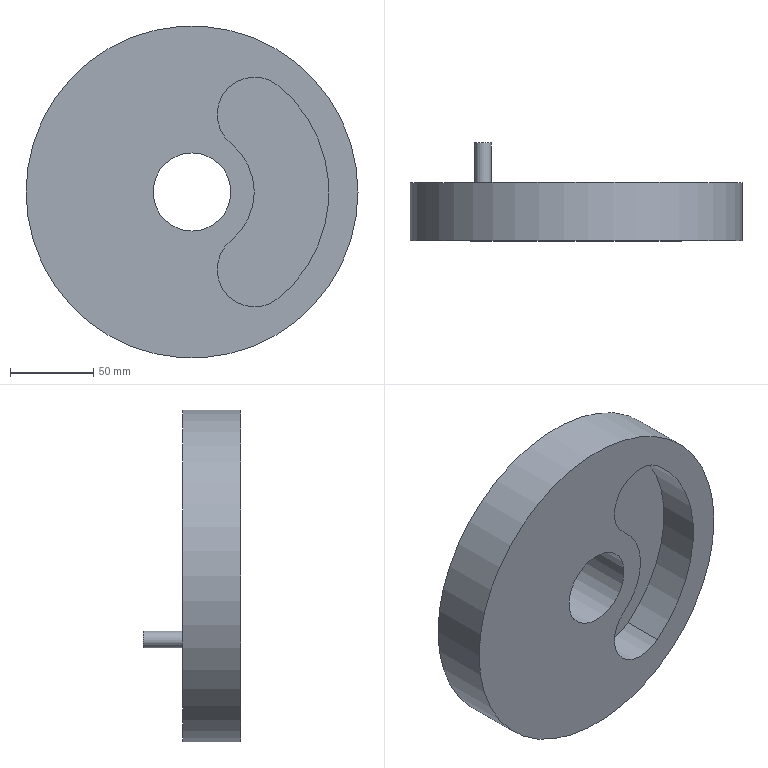Component | NX | TURNTABLE | 1 solid | 11 faces | box 200 x 59 x 200 mm | volume 880594 mm3 | cylinder 7 | plane 4 | commonest cylinder face diameters 45 x2 165 x1 47 x1 200 x1 75 x1 10 x1
STEP:
#1=CARTESIAN_POINT('',(0.,0.,0.));
#2=DIRECTION('',(0.,0.,1.));
#3=DIRECTION('',(1.,0.,0.));
#4=AXIS2_PLACEMENT_3D('',#1,#2,#3);
#5=CARTESIAN_POINT('',(23.557,-35.,29.178));
#6=VERTEX_POINT('',#5);
#7=CARTESIAN_POINT('',(23.557,-10.,29.178));
#8=VERTEX_POINT('',#7);
#9=CARTESIAN_POINT('',(23.557,-35.,29.178));
#10=DIRECTION('',(0.,1.,0.));
#11=VECTOR('',#10,1.);
#12=LINE('',#9,#11);
#13=CARTESIAN_POINT('',(37.691,-35.,46.684));
#14=DIRECTION('',(0.,1.,0.));
#15=DIRECTION('',(0.,0.,1.));
#16=AXIS2_PLACEMENT_3D('',#13,#14,#15);
#17=CYLINDRICAL_SURFACE('',#16,22.5);
#18=CARTESIAN_POINT('',(3.821,0.));
#19=DIRECTION('',(0.,1.));
#20=VECTOR('',#19,1.);
#21=LINE('',#18,#20);
#22=(GEOMETRIC_REPRESENTATION_CONTEXT(2)PARAMETRIC_REPRESENTATION_CONTEXT()REPRESENTATION_CONTEXT('',''));
#23=DEFINITIONAL_REPRESENTATION('',(#21),#22);
#24=PCURVE('',#17,#23);
#25=CARTESIAN_POINT('',(0.,-35.,0.));
#26=DIRECTION('',(0.,1.,0.));
#27=DIRECTION('',(0.,0.,1.));
#28=AXIS2_PLACEMENT_3D('',#25,#26,#27);
#29=CYLINDRICAL_SURFACE('',#28,37.5);
#30=CARTESIAN_POINT('',(0.6792,0.));
#31=DIRECTION('',(0.,1.));
#32=VECTOR('',#31,1.);
#33=LINE('',#30,#32);
#34=(GEOMETRIC_REPRESENTATION_CONTEXT(2)PARAMETRIC_REPRESENTATION_CONTEXT()REPRESENTATION_CONTEXT('',''));
#35=DEFINITIONAL_REPRESENTATION('',(#33),#34);
#36=PCURVE('',#29,#35);
#37=SURFACE_CURVE('',#12,(#24,#36),.PCURVE_S1.);
#38=EDGE_CURVE('',#6,#8,#37,.T.);
#39=ORIENTED_EDGE('',*,*,#38,.F.);
#40=CARTESIAN_POINT('',(51.825,-35.,64.191));
#41=VERTEX_POINT('',#40);
#42=CARTESIAN_POINT('',(37.691,-35.,46.684));
#43=DIRECTION('',(0.,-1.,0.));
#44=DIRECTION('',(0.7193,0.,-0.6947));
#45=AXIS2_PLACEMENT_3D('',#42,#43,#44);
#46=CIRCLE('',#45,22.5);
#47=CARTESIAN_POINT('',(8.622,0.));
#48=DIRECTION('',(-1.,0.));
#49=VECTOR('',#48,1.);
#50=LINE('',#47,#49);
#51=(GEOMETRIC_REPRESENTATION_CONTEXT(2)PARAMETRIC_REPRESENTATION_CONTEXT()REPRESENTATION_CONTEXT('',''));
#52=DEFINITIONAL_REPRESENTATION('',(#50),#51);
#53=PCURVE('',#17,#52);
#54=CARTESIAN_POINT('',(12.564,-35.,15.561));
#55=DIRECTION('',(0.,-1.,0.));
#56=DIRECTION('',(0.,0.,-1.));
#57=AXIS2_PLACEMENT_3D('',#54,#55,#56);
#58=PLANE('',#57);
#59=CARTESIAN_POINT('',(-31.123,25.127));
#60=DIRECTION('',(0.6947,0.7193));
#61=AXIS2_PLACEMENT_2D('',#59,#60);
#62=CIRCLE('',#61,22.5);
#63=(GEOMETRIC_REPRESENTATION_CONTEXT(2)PARAMETRIC_REPRESENTATION_CONTEXT()REPRESENTATION_CONTEXT('',''));
#64=DEFINITIONAL_REPRESENTATION('',(#62),#63);
#65=PCURVE('',#58,#64);
#66=SURFACE_CURVE('',#46,(#53,#65),.PCURVE_S1.);
#67=EDGE_CURVE('',#41,#6,#66,.T.);
#68=ORIENTED_EDGE('',*,*,#67,.F.);
#69=CARTESIAN_POINT('',(51.825,-10.,64.191));
#70=VERTEX_POINT('',#69);
#71=CARTESIAN_POINT('',(51.825,-35.,64.191));
#72=DIRECTION('',(0.,1.,0.));
#73=VECTOR('',#72,1.);
#74=LINE('',#71,#73);
#75=CARTESIAN_POINT('',(6.962,0.));
#76=DIRECTION('',(0.,1.));
#77=VECTOR('',#76,1.);
#78=LINE('',#75,#77);
#79=(GEOMETRIC_REPRESENTATION_CONTEXT(2)PARAMETRIC_REPRESENTATION_CONTEXT()REPRESENTATION_CONTEXT('',''));
#80=DEFINITIONAL_REPRESENTATION('',(#78),#79);
#81=PCURVE('',#17,#80);
#82=CARTESIAN_POINT('',(0.,-35.,0.));
#83=DIRECTION('',(0.,1.,0.));
#84=DIRECTION('',(0.,0.,1.));
#85=AXIS2_PLACEMENT_3D('',#82,#83,#84);
#86=CYLINDRICAL_SURFACE('',#85,82.5);
#87=CARTESIAN_POINT('',(0.6792,0.));
#88=DIRECTION('',(0.,1.));
#89=VECTOR('',#88,1.);
#90=LINE('',#87,#89);
#91=(GEOMETRIC_REPRESENTATION_CONTEXT(2)PARAMETRIC_REPRESENTATION_CONTEXT()REPRESENTATION_CONTEXT('',''));
#92=DEFINITIONAL_REPRESENTATION('',(#90),#91);
#93=PCURVE('',#86,#92);
#94=SURFACE_CURVE('',#74,(#81,#93),.PCURVE_S1.);
#95=EDGE_CURVE('',#41,#70,#94,.T.);
#96=ORIENTED_EDGE('',*,*,#95,.T.);
#97=CARTESIAN_POINT('',(37.691,-10.,46.684));
#98=DIRECTION('',(0.,-1.,0.));
#99=DIRECTION('',(0.7193,0.,-0.6947));
#100=AXIS2_PLACEMENT_3D('',#97,#98,#99);
#101=CIRCLE('',#100,22.5);
#102=CARTESIAN_POINT('',(8.622,25.));
#103=DIRECTION('',(-1.,0.));
#104=VECTOR('',#103,1.);
#105=LINE('',#102,#104);
#106=(GEOMETRIC_REPRESENTATION_CONTEXT(2)PARAMETRIC_REPRESENTATION_CONTEXT()REPRESENTATION_CONTEXT('',''));
#107=DEFINITIONAL_REPRESENTATION('',(#105),#106);
#108=PCURVE('',#17,#107);
#109=CARTESIAN_POINT('',(18.845,-10.,23.342));
#110=DIRECTION('',(0.,-1.,0.));
#111=DIRECTION('',(0.,0.,-1.));
#112=AXIS2_PLACEMENT_3D('',#109,#110,#111);
#113=PLANE('',#112);
#114=CARTESIAN_POINT('',(-23.342,18.845));
#115=DIRECTION('',(0.6947,0.7193));
#116=AXIS2_PLACEMENT_2D('',#114,#115);
#117=CIRCLE('',#116,22.5);
#118=(GEOMETRIC_REPRESENTATION_CONTEXT(2)PARAMETRIC_REPRESENTATION_CONTEXT()REPRESENTATION_CONTEXT('',''));
#119=DEFINITIONAL_REPRESENTATION('',(#117),#118);
#120=PCURVE('',#113,#119);
#121=SURFACE_CURVE('',#101,(#108,#120),.PCURVE_S1.);
#122=EDGE_CURVE('',#70,#8,#121,.T.);
#123=ORIENTED_EDGE('',*,*,#122,.T.);
#124=EDGE_LOOP('',(#39,#68,#96,#123));
#125=FACE_BOUND('',#124,.F.);
#126=ADVANCED_FACE('',(#125),#17,.F.);
#127=ORIENTED_EDGE('',*,*,#95,.F.);
#128=CARTESIAN_POINT('',(51.825,-35.,-64.191));
#129=VERTEX_POINT('',#128);
#130=CARTESIAN_POINT('',(0.,-35.,0.));
#131=DIRECTION('',(0.,-1.,0.));
#132=DIRECTION('',(1.,0.,-0.));
#133=AXIS2_PLACEMENT_3D('',#130,#131,#132);
#134=CIRCLE('',#133,82.5);
#135=CARTESIAN_POINT('',(7.854,0.));
#136=DIRECTION('',(-1.,0.));
#137=VECTOR('',#136,1.);
#138=LINE('',#135,#137);
#139=(GEOMETRIC_REPRESENTATION_CONTEXT(2)PARAMETRIC_REPRESENTATION_CONTEXT()REPRESENTATION_CONTEXT('',''));
#140=DEFINITIONAL_REPRESENTATION('',(#138),#139);
#141=PCURVE('',#86,#140);
#142=CARTESIAN_POINT('',(15.561,-12.564));
#143=DIRECTION('',(0.,1.));
#144=AXIS2_PLACEMENT_2D('',#142,#143);
#145=CIRCLE('',#144,82.5);
#146=(GEOMETRIC_REPRESENTATION_CONTEXT(2)PARAMETRIC_REPRESENTATION_CONTEXT()REPRESENTATION_CONTEXT('',''));
#147=DEFINITIONAL_REPRESENTATION('',(#145),#146);
#148=PCURVE('',#58,#147);
#149=SURFACE_CURVE('',#134,(#141,#148),.PCURVE_S1.);
#150=EDGE_CURVE('',#129,#41,#149,.T.);
#151=ORIENTED_EDGE('',*,*,#150,.F.);
#152=CARTESIAN_POINT('',(51.825,-10.,-64.191));
#153=VERTEX_POINT('',#152);
#154=CARTESIAN_POINT('',(51.825,-35.,-64.191));
#155=DIRECTION('',(0.,1.,0.));
#156=VECTOR('',#155,1.);
#157=LINE('',#154,#156);
#158=CARTESIAN_POINT('',(2.462,0.));
#159=DIRECTION('',(0.,1.));
#160=VECTOR('',#159,1.);
#161=LINE('',#158,#160);
#162=(GEOMETRIC_REPRESENTATION_CONTEXT(2)PARAMETRIC_REPRESENTATION_CONTEXT()REPRESENTATION_CONTEXT('',''));
#163=DEFINITIONAL_REPRESENTATION('',(#161),#162);
#164=PCURVE('',#86,#163);
#165=CARTESIAN_POINT('',(37.691,-35.,-46.684));
#166=DIRECTION('',(0.,1.,0.));
#167=DIRECTION('',(0.,0.,1.));
#168=AXIS2_PLACEMENT_3D('',#165,#166,#167);
#169=CYLINDRICAL_SURFACE('',#168,22.5);
#170=CARTESIAN_POINT('',(2.462,0.));
#171=DIRECTION('',(0.,1.));
#172=VECTOR('',#171,1.);
#173=LINE('',#170,#172);
#174=(GEOMETRIC_REPRESENTATION_CONTEXT(2)PARAMETRIC_REPRESENTATION_CONTEXT()REPRESENTATION_CONTEXT('',''));
#175=DEFINITIONAL_REPRESENTATION('',(#173),#174);
#176=PCURVE('',#169,#175);
#177=SURFACE_CURVE('',#157,(#164,#176),.PCURVE_S1.);
#178=EDGE_CURVE('',#129,#153,#177,.T.);
#179=ORIENTED_EDGE('',*,*,#178,.T.);
#180=CARTESIAN_POINT('',(0.,-10.,0.));
#181=DIRECTION('',(0.,-1.,0.));
#182=DIRECTION('',(1.,0.,-0.));
#183=AXIS2_PLACEMENT_3D('',#180,#181,#182);
#184=CIRCLE('',#183,82.5);
#185=CARTESIAN_POINT('',(7.854,25.));
#186=DIRECTION('',(-1.,0.));
#187=VECTOR('',#186,1.);
#188=LINE('',#185,#187);
#189=(GEOMETRIC_REPRESENTATION_CONTEXT(2)PARAMETRIC_REPRESENTATION_CONTEXT()REPRESENTATION_CONTEXT('',''));
#190=DEFINITIONAL_REPRESENTATION('',(#188),#189);
#191=PCURVE('',#86,#190);
#192=CARTESIAN_POINT('',(23.342,-18.845));
#193=DIRECTION('',(0.,1.));
#194=AXIS2_PLACEMENT_2D('',#192,#193);
#195=CIRCLE('',#194,82.5);
#196=(GEOMETRIC_REPRESENTATION_CONTEXT(2)PARAMETRIC_REPRESENTATION_CONTEXT()REPRESENTATION_CONTEXT('',''));
#197=DEFINITIONAL_REPRESENTATION('',(#195),#196);
#198=PCURVE('',#113,#197);
#199=SURFACE_CURVE('',#184,(#191,#198),.PCURVE_S1.);
#200=EDGE_CURVE('',#153,#70,#199,.T.);
#201=ORIENTED_EDGE('',*,*,#200,.T.);
#202=EDGE_LOOP('',(#127,#151,#179,#201));
#203=FACE_BOUND('',#202,.F.);
#204=ADVANCED_FACE('',(#203),#86,.F.);
#205=ORIENTED_EDGE('',*,*,#178,.F.);
#206=CARTESIAN_POINT('',(23.557,-35.,-29.178));
#207=VERTEX_POINT('',#206);
#208=CARTESIAN_POINT('',(37.691,-35.,-46.684));
#209=DIRECTION('',(0.,-1.,0.));
#210=DIRECTION('',(1.,0.,0.));
#211=AXIS2_PLACEMENT_3D('',#208,#209,#210);
#212=CIRCLE('',#211,22.5);
#213=CARTESIAN_POINT('',(7.854,0.));
#214=DIRECTION('',(-1.,0.));
#215=VECTOR('',#214,1.);
#216=LINE('',#213,#215);
#217=(GEOMETRIC_REPRESENTATION_CONTEXT(2)PARAMETRIC_REPRESENTATION_CONTEXT()REPRESENTATION_CONTEXT('',''));
#218=DEFINITIONAL_REPRESENTATION('',(#216),#217);
#219=PCURVE('',#169,#218);
#220=CARTESIAN_POINT('',(62.246,25.127));
#221=DIRECTION('',(0.,1.));
#222=AXIS2_PLACEMENT_2D('',#220,#221);
#223=CIRCLE('',#222,22.5);
#224=(GEOMETRIC_REPRESENTATION_CONTEXT(2)PARAMETRIC_REPRESENTATION_CONTEXT()REPRESENTATION_CONTEXT('',''));
#225=DEFINITIONAL_REPRESENTATION('',(#223),#224);
#226=PCURVE('',#58,#225);
#227=SURFACE_CURVE('',#212,(#219,#226),.PCURVE_S1.);
#228=EDGE_CURVE('',#207,#129,#227,.T.);
#229=ORIENTED_EDGE('',*,*,#228,.F.);
#230=CARTESIAN_POINT('',(23.557,-10.,-29.178));
#231=VERTEX_POINT('',#230);
#232=CARTESIAN_POINT('',(23.557,-35.,-29.178));
#233=DIRECTION('',(0.,1.,0.));
#234=VECTOR('',#233,1.);
#235=LINE('',#232,#234);
#236=CARTESIAN_POINT('',(5.604,0.));
#237=DIRECTION('',(0.,1.));
#238=VECTOR('',#237,1.);
#239=LINE('',#236,#238);
#240=(GEOMETRIC_REPRESENTATION_CONTEXT(2)PARAMETRIC_REPRESENTATION_CONTEXT()REPRESENTATION_CONTEXT('',''));
#241=DEFINITIONAL_REPRESENTATION('',(#239),#240);
#242=PCURVE('',#169,#241);
#243=CARTESIAN_POINT('',(2.462,0.));
#244=DIRECTION('',(0.,1.));
#245=VECTOR('',#244,1.);
#246=LINE('',#243,#245);
#247=(GEOMETRIC_REPRESENTATION_CONTEXT(2)PARAMETRIC_REPRESENTATION_CONTEXT()REPRESENTATION_CONTEXT('',''));
#248=DEFINITIONAL_REPRESENTATION('',(#246),#247);
#249=PCURVE('',#29,#248);
#250=SURFACE_CURVE('',#235,(#242,#249),.PCURVE_S1.);
#251=EDGE_CURVE('',#207,#231,#250,.T.);
#252=ORIENTED_EDGE('',*,*,#251,.T.);
#253=CARTESIAN_POINT('',(37.691,-10.,-46.684));
#254=DIRECTION('',(0.,-1.,0.));
#255=DIRECTION('',(1.,0.,0.));
#256=AXIS2_PLACEMENT_3D('',#253,#254,#255);
#257=CIRCLE('',#256,22.5);
#258=CARTESIAN_POINT('',(7.854,25.));
#259=DIRECTION('',(-1.,0.));
#260=VECTOR('',#259,1.);
#261=LINE('',#258,#260);
#262=(GEOMETRIC_REPRESENTATION_CONTEXT(2)PARAMETRIC_REPRESENTATION_CONTEXT()REPRESENTATION_CONTEXT('',''));
#263=DEFINITIONAL_REPRESENTATION('',(#261),#262);
#264=PCURVE('',#169,#263);
#265=CARTESIAN_POINT('',(70.026,18.845));
#266=DIRECTION('',(0.,1.));
#267=AXIS2_PLACEMENT_2D('',#265,#266);
#268=CIRCLE('',#267,22.5);
#269=(GEOMETRIC_REPRESENTATION_CONTEXT(2)PARAMETRIC_REPRESENTATION_CONTEXT()REPRESENTATION_CONTEXT('',''));
#270=DEFINITIONAL_REPRESENTATION('',(#268),#269);
#271=PCURVE('',#113,#270);
#272=SURFACE_CURVE('',#257,(#264,#271),.PCURVE_S1.);
#273=EDGE_CURVE('',#231,#153,#272,.T.);
#274=ORIENTED_EDGE('',*,*,#273,.T.);
#275=EDGE_LOOP('',(#205,#229,#252,#274));
#276=FACE_BOUND('',#275,.F.);
#277=ADVANCED_FACE('',(#276),#169,.F.);
#278=CARTESIAN_POINT('',(0.,-35.,-23.5));
#279=VERTEX_POINT('',#278);
#280=CARTESIAN_POINT('',(0.,-35.,0.));
#281=DIRECTION('',(0.,-1.,0.));
#282=DIRECTION('',(0.,0.,-1.));
#283=AXIS2_PLACEMENT_3D('',#280,#281,#282);
#284=CIRCLE('',#283,23.5);
#285=CARTESIAN_POINT('',(0.,-35.,0.));
#286=DIRECTION('',(0.,1.,0.));
#287=DIRECTION('',(0.,0.,1.));
#288=AXIS2_PLACEMENT_3D('',#285,#286,#287);
#289=CYLINDRICAL_SURFACE('',#288,23.5);
#290=CARTESIAN_POINT('',(9.425,0.));
#291=DIRECTION('',(-1.,0.));
#292=VECTOR('',#291,1.);
#293=LINE('',#290,#292);
#294=(GEOMETRIC_REPRESENTATION_CONTEXT(2)PARAMETRIC_REPRESENTATION_CONTEXT()REPRESENTATION_CONTEXT('',''));
#295=DEFINITIONAL_REPRESENTATION('',(#293),#294);
#296=PCURVE('',#289,#295);
#297=CARTESIAN_POINT('',(15.561,-12.564));
#298=DIRECTION('',(1.,0.));
#299=AXIS2_PLACEMENT_2D('',#297,#298);
#300=CIRCLE('',#299,23.5);
#301=(GEOMETRIC_REPRESENTATION_CONTEXT(2)PARAMETRIC_REPRESENTATION_CONTEXT()REPRESENTATION_CONTEXT('',''));
#302=DEFINITIONAL_REPRESENTATION('',(#300),#301);
#303=PCURVE('',#58,#302);
#304=SURFACE_CURVE('',#284,(#296,#303),.PCURVE_S1.);
#305=EDGE_CURVE('',#279,#279,#304,.T.);
#306=ORIENTED_EDGE('',*,*,#305,.F.);
#307=CARTESIAN_POINT('',(0.,0.,-23.5));
#308=VERTEX_POINT('',#307);
#309=CARTESIAN_POINT('',(0.,-35.,-23.5));
#310=CARTESIAN_POINT('',(0.,0.,-23.5));
#311=B_SPLINE_CURVE_WITH_KNOTS('',1,(#309,#310),.UNSPECIFIED.,.F.,.F.,(2,2),(0.,35.),.PIECEWISE_BEZIER_KNOTS.);
#312=CARTESIAN_POINT('',(9.425,0.));
#313=DIRECTION('',(0.,1.));
#314=VECTOR('',#313,1.);
#315=LINE('',#312,#314);
#316=(GEOMETRIC_REPRESENTATION_CONTEXT(2)PARAMETRIC_REPRESENTATION_CONTEXT()REPRESENTATION_CONTEXT('',''));
#317=DEFINITIONAL_REPRESENTATION('',(#315),#316);
#318=PCURVE('',#289,#317);
#319=CARTESIAN_POINT('',(3.142,0.));
#320=DIRECTION('',(0.,1.));
#321=VECTOR('',#320,1.);
#322=LINE('',#319,#321);
#323=(GEOMETRIC_REPRESENTATION_CONTEXT(2)PARAMETRIC_REPRESENTATION_CONTEXT()REPRESENTATION_CONTEXT('',''));
#324=DEFINITIONAL_REPRESENTATION('',(#322),#323);
#325=PCURVE('',#289,#324);
#326=SEAM_CURVE('',#311,(#318,#325),.PCURVE_S1.);
#327=EDGE_CURVE('',#279,#308,#326,.T.);
#328=ORIENTED_EDGE('',*,*,#327,.T.);
#329=CARTESIAN_POINT('',(0.,0.,0.));
#330=DIRECTION('',(0.,-1.,0.));
#331=DIRECTION('',(0.,0.,-1.));
#332=AXIS2_PLACEMENT_3D('',#329,#330,#331);
#333=CIRCLE('',#332,23.5);
#334=CARTESIAN_POINT('',(9.425,35.));
#335=DIRECTION('',(-1.,0.));
#336=VECTOR('',#335,1.);
#337=LINE('',#334,#336);
#338=(GEOMETRIC_REPRESENTATION_CONTEXT(2)PARAMETRIC_REPRESENTATION_CONTEXT()REPRESENTATION_CONTEXT('',''));
#339=DEFINITIONAL_REPRESENTATION('',(#337),#338);
#340=PCURVE('',#289,#339);
#341=CARTESIAN_POINT('',(12.564,0.,15.561));
#342=DIRECTION('',(0.,-1.,0.));
#343=DIRECTION('',(0.,0.,-1.));
#344=AXIS2_PLACEMENT_3D('',#341,#342,#343);
#345=PLANE('',#344);
#346=CARTESIAN_POINT('',(15.561,-12.564));
#347=DIRECTION('',(1.,0.));
#348=AXIS2_PLACEMENT_2D('',#346,#347);
#349=CIRCLE('',#348,23.5);
#350=(GEOMETRIC_REPRESENTATION_CONTEXT(2)PARAMETRIC_REPRESENTATION_CONTEXT()REPRESENTATION_CONTEXT('',''));
#351=DEFINITIONAL_REPRESENTATION('',(#349),#350);
#352=PCURVE('',#345,#351);
#353=SURFACE_CURVE('',#333,(#340,#352),.PCURVE_S1.);
#354=EDGE_CURVE('',#308,#308,#353,.T.);
#355=ORIENTED_EDGE('',*,*,#354,.T.);
#356=ORIENTED_EDGE('',*,*,#327,.F.);
#357=EDGE_LOOP('',(#306,#328,#355,#356));
#358=FACE_BOUND('',#357,.F.);
#359=ADVANCED_FACE('',(#358),#289,.F.);
#360=CARTESIAN_POINT('',(100.,-35.,-0.));
#361=VERTEX_POINT('',#360);
#362=CARTESIAN_POINT('',(0.,-35.,0.));
#363=DIRECTION('',(0.,-1.,0.));
#364=DIRECTION('',(1.,0.,-0.));
#365=AXIS2_PLACEMENT_3D('',#362,#363,#364);
#366=CIRCLE('',#365,100.);
#367=CARTESIAN_POINT('',(0.,-35.,0.));
#368=DIRECTION('',(0.,1.,0.));
#369=DIRECTION('',(0.,0.,1.));
#370=AXIS2_PLACEMENT_3D('',#367,#368,#369);
#371=CYLINDRICAL_SURFACE('',#370,100.);
#372=CARTESIAN_POINT('',(7.854,0.));
#373=DIRECTION('',(-1.,0.));
#374=VECTOR('',#373,1.);
#375=LINE('',#372,#374);
#376=(GEOMETRIC_REPRESENTATION_CONTEXT(2)PARAMETRIC_REPRESENTATION_CONTEXT()REPRESENTATION_CONTEXT('',''));
#377=DEFINITIONAL_REPRESENTATION('',(#375),#376);
#378=PCURVE('',#371,#377);
#379=CARTESIAN_POINT('',(15.561,-12.564));
#380=DIRECTION('',(0.,1.));
#381=AXIS2_PLACEMENT_2D('',#379,#380);
#382=CIRCLE('',#381,100.);
#383=(GEOMETRIC_REPRESENTATION_CONTEXT(2)PARAMETRIC_REPRESENTATION_CONTEXT()REPRESENTATION_CONTEXT('',''));
#384=DEFINITIONAL_REPRESENTATION('',(#382),#383);
#385=PCURVE('',#58,#384);
#386=SURFACE_CURVE('',#366,(#378,#385),.PCURVE_S1.);
#387=EDGE_CURVE('',#361,#361,#386,.T.);
#388=ORIENTED_EDGE('',*,*,#387,.F.);
#389=CARTESIAN_POINT('',(100.,0.,-0.));
#390=VERTEX_POINT('',#389);
#391=CARTESIAN_POINT('',(100.,-35.,0.));
#392=CARTESIAN_POINT('',(100.,0.,0.));
#393=B_SPLINE_CURVE_WITH_KNOTS('',1,(#391,#392),.UNSPECIFIED.,.F.,.F.,(2,2),(0.,35.),.PIECEWISE_BEZIER_KNOTS.);
#394=CARTESIAN_POINT('',(7.854,0.));
#395=DIRECTION('',(0.,1.));
#396=VECTOR('',#395,1.);
#397=LINE('',#394,#396);
#398=(GEOMETRIC_REPRESENTATION_CONTEXT(2)PARAMETRIC_REPRESENTATION_CONTEXT()REPRESENTATION_CONTEXT('',''));
#399=DEFINITIONAL_REPRESENTATION('',(#397),#398);
#400=PCURVE('',#371,#399);
#401=CARTESIAN_POINT('',(1.571,0.));
#402=DIRECTION('',(0.,1.));
#403=VECTOR('',#402,1.);
#404=LINE('',#401,#403);
#405=(GEOMETRIC_REPRESENTATION_CONTEXT(2)PARAMETRIC_REPRESENTATION_CONTEXT()REPRESENTATION_CONTEXT('',''));
#406=DEFINITIONAL_REPRESENTATION('',(#404),#405);
#407=PCURVE('',#371,#406);
#408=SEAM_CURVE('',#393,(#400,#407),.PCURVE_S1.);
#409=EDGE_CURVE('',#361,#390,#408,.T.);
#410=ORIENTED_EDGE('',*,*,#409,.T.);
#411=CARTESIAN_POINT('',(0.,0.,0.));
#412=DIRECTION('',(0.,-1.,0.));
#413=DIRECTION('',(1.,0.,-0.));
#414=AXIS2_PLACEMENT_3D('',#411,#412,#413);
#415=CIRCLE('',#414,100.);
#416=CARTESIAN_POINT('',(7.854,35.));
#417=DIRECTION('',(-1.,0.));
#418=VECTOR('',#417,1.);
#419=LINE('',#416,#418);
#420=(GEOMETRIC_REPRESENTATION_CONTEXT(2)PARAMETRIC_REPRESENTATION_CONTEXT()REPRESENTATION_CONTEXT('',''));
#421=DEFINITIONAL_REPRESENTATION('',(#419),#420);
#422=PCURVE('',#371,#421);
#423=CARTESIAN_POINT('',(15.561,-12.564));
#424=DIRECTION('',(0.,1.));
#425=AXIS2_PLACEMENT_2D('',#423,#424);
#426=CIRCLE('',#425,100.);
#427=(GEOMETRIC_REPRESENTATION_CONTEXT(2)PARAMETRIC_REPRESENTATION_CONTEXT()REPRESENTATION_CONTEXT('',''));
#428=DEFINITIONAL_REPRESENTATION('',(#426),#427);
#429=PCURVE('',#345,#428);
#430=SURFACE_CURVE('',#415,(#422,#429),.PCURVE_S1.);
#431=EDGE_CURVE('',#390,#390,#430,.T.);
#432=ORIENTED_EDGE('',*,*,#431,.T.);
#433=ORIENTED_EDGE('',*,*,#409,.F.);
#434=EDGE_LOOP('',(#388,#410,#432,#433));
#435=FACE_BOUND('',#434,.T.);
#436=ADVANCED_FACE('',(#435),#371,.T.);
#437=CARTESIAN_POINT('',(0.,-10.,0.));
#438=DIRECTION('',(0.,1.,0.));
#439=DIRECTION('',(1.,0.,0.));
#440=AXIS2_PLACEMENT_3D('',#437,#438,#439);
#441=CIRCLE('',#440,37.5);
#442=CARTESIAN_POINT('',(-4.712,25.));
#443=DIRECTION('',(1.,0.));
#444=VECTOR('',#443,1.);
#445=LINE('',#442,#444);
#446=(GEOMETRIC_REPRESENTATION_CONTEXT(2)PARAMETRIC_REPRESENTATION_CONTEXT()REPRESENTATION_CONTEXT('',''));
#447=DEFINITIONAL_REPRESENTATION('',(#445),#446);
#448=PCURVE('',#29,#447);
#449=CARTESIAN_POINT('',(23.342,18.655));
#450=CARTESIAN_POINT('',(88.294,18.655));
#451=CARTESIAN_POINT('',(55.818,-37.595));
#452=CARTESIAN_POINT('',(23.342,-93.845));
#453=CARTESIAN_POINT('',(-9.134,-37.595));
#454=CARTESIAN_POINT('',(-41.61,18.655));
#455=CARTESIAN_POINT('',(23.342,18.655));
#456=(BOUNDED_CURVE()B_SPLINE_CURVE(2,(#449,#450,#451,#452,#453,#454,#455),.UNSPECIFIED.,.T.,.F.)B_SPLINE_CURVE_WITH_KNOTS((1,2,2,2,2,1),(-2.094,0.,2.094,4.189,6.283,8.378),.UNSPECIFIED.)CURVE()GEOMETRIC_REPRESENTATION_ITEM()RATIONAL_B_SPLINE_CURVE((1.,0.5,1.,0.5,1.,0.5,1.))REPRESENTATION_ITEM(''));
#457=(GEOMETRIC_REPRESENTATION_CONTEXT(2)PARAMETRIC_REPRESENTATION_CONTEXT()REPRESENTATION_CONTEXT('',''));
#458=DEFINITIONAL_REPRESENTATION('',(#456),#457);
#459=PCURVE('',#113,#458);
#460=SURFACE_CURVE('',#441,(#448,#459),.PCURVE_S1.);
#461=EDGE_CURVE('',#8,#231,#460,.T.);
#462=ORIENTED_EDGE('',*,*,#461,.F.);
#463=ORIENTED_EDGE('',*,*,#38,.F.);
#464=CARTESIAN_POINT('',(0.,-35.,0.));
#465=DIRECTION('',(0.,1.,0.));
#466=DIRECTION('',(1.,0.,0.));
#467=AXIS2_PLACEMENT_3D('',#464,#465,#466);
#468=CIRCLE('',#467,37.5);
#469=CARTESIAN_POINT('',(-4.712,0.));
#470=DIRECTION('',(1.,0.));
#471=VECTOR('',#470,1.);
#472=LINE('',#469,#471);
#473=(GEOMETRIC_REPRESENTATION_CONTEXT(2)PARAMETRIC_REPRESENTATION_CONTEXT()REPRESENTATION_CONTEXT('',''));
#474=DEFINITIONAL_REPRESENTATION('',(#472),#473);
#475=PCURVE('',#29,#474);
#476=CARTESIAN_POINT('',(15.561,24.936));
#477=CARTESIAN_POINT('',(80.513,24.936));
#478=CARTESIAN_POINT('',(48.037,-31.314));
#479=CARTESIAN_POINT('',(15.561,-87.564));
#480=CARTESIAN_POINT('',(-16.915,-31.314));
#481=CARTESIAN_POINT('',(-49.39,24.936));
#482=CARTESIAN_POINT('',(15.561,24.936));
#483=(BOUNDED_CURVE()B_SPLINE_CURVE(2,(#476,#477,#478,#479,#480,#481,#482),.UNSPECIFIED.,.T.,.F.)B_SPLINE_CURVE_WITH_KNOTS((1,2,2,2,2,1),(-2.094,0.,2.094,4.189,6.283,8.378),.UNSPECIFIED.)CURVE()GEOMETRIC_REPRESENTATION_ITEM()RATIONAL_B_SPLINE_CURVE((1.,0.5,1.,0.5,1.,0.5,1.))REPRESENTATION_ITEM(''));
#484=(GEOMETRIC_REPRESENTATION_CONTEXT(2)PARAMETRIC_REPRESENTATION_CONTEXT()REPRESENTATION_CONTEXT('',''));
#485=DEFINITIONAL_REPRESENTATION('',(#483),#484);
#486=PCURVE('',#58,#485);
#487=SURFACE_CURVE('',#468,(#475,#486),.PCURVE_S1.);
#488=EDGE_CURVE('',#6,#207,#487,.T.);
#489=ORIENTED_EDGE('',*,*,#488,.T.);
#490=ORIENTED_EDGE('',*,*,#251,.T.);
#491=EDGE_LOOP('',(#462,#463,#489,#490));
#492=FACE_BOUND('',#491,.T.);
#493=ADVANCED_FACE('',(#492),#29,.T.);
#494=ORIENTED_EDGE('',*,*,#387,.T.);
#495=EDGE_LOOP('',(#494));
#496=FACE_BOUND('',#495,.T.);
#497=ORIENTED_EDGE('',*,*,#305,.F.);
#498=EDGE_LOOP('',(#497));
#499=FACE_BOUND('',#498,.T.);
#500=ORIENTED_EDGE('',*,*,#67,.F.);
#501=ORIENTED_EDGE('',*,*,#150,.F.);
#502=ORIENTED_EDGE('',*,*,#228,.F.);
#503=ORIENTED_EDGE('',*,*,#488,.F.);
#504=EDGE_LOOP('',(#500,#501,#502,#503));
#505=FACE_BOUND('',#504,.T.);
#506=ADVANCED_FACE('',(#496,#499,#505),#58,.T.);
#507=CARTESIAN_POINT('',(-61.175,0.,-38.332));
#508=VERTEX_POINT('',#507);
#509=CARTESIAN_POINT('',(-56.175,0.,-38.332));
#510=DIRECTION('',(0.,-1.,0.));
#511=DIRECTION('',(-1.,0.,0.));
#512=AXIS2_PLACEMENT_3D('',#509,#510,#511);
#513=CIRCLE('',#512,5.);
#514=CARTESIAN_POINT('',(53.893,-68.739));
#515=DIRECTION('',(0.,-1.));
#516=AXIS2_PLACEMENT_2D('',#514,#515);
#517=CIRCLE('',#516,5.);
#518=(GEOMETRIC_REPRESENTATION_CONTEXT(2)PARAMETRIC_REPRESENTATION_CONTEXT()REPRESENTATION_CONTEXT('',''));
#519=DEFINITIONAL_REPRESENTATION('',(#517),#518);
#520=PCURVE('',#345,#519);
#521=CARTESIAN_POINT('',(-56.175,24.,-38.332));
#522=DIRECTION('',(0.,-1.,0.));
#523=DIRECTION('',(0.,0.,-1.));
#524=AXIS2_PLACEMENT_3D('',#521,#522,#523);
#525=CYLINDRICAL_SURFACE('',#524,5.);
#526=CARTESIAN_POINT('',(4.712,24.));
#527=DIRECTION('',(1.,0.));
#528=VECTOR('',#527,1.);
#529=LINE('',#526,#528);
#530=(GEOMETRIC_REPRESENTATION_CONTEXT(2)PARAMETRIC_REPRESENTATION_CONTEXT()REPRESENTATION_CONTEXT('',''));
#531=DEFINITIONAL_REPRESENTATION('',(#529),#530);
#532=PCURVE('',#525,#531);
#533=SURFACE_CURVE('',#513,(#520,#532),.PCURVE_S1.);
#534=EDGE_CURVE('',#508,#508,#533,.T.);
#535=ORIENTED_EDGE('',*,*,#534,.T.);
#536=EDGE_LOOP('',(#535));
#537=FACE_BOUND('',#536,.T.);
#538=ORIENTED_EDGE('',*,*,#431,.F.);
#539=EDGE_LOOP('',(#538));
#540=FACE_BOUND('',#539,.T.);
#541=ORIENTED_EDGE('',*,*,#354,.T.);
#542=EDGE_LOOP('',(#541));
#543=FACE_BOUND('',#542,.T.);
#544=ADVANCED_FACE('',(#537,#540,#543),#345,.F.);
#545=ORIENTED_EDGE('',*,*,#122,.T.);
#546=ORIENTED_EDGE('',*,*,#461,.T.);
#547=ORIENTED_EDGE('',*,*,#273,.T.);
#548=ORIENTED_EDGE('',*,*,#200,.T.);
#549=EDGE_LOOP('',(#545,#546,#547,#548));
#550=FACE_BOUND('',#549,.T.);
#551=ADVANCED_FACE('',(#550),#113,.T.);
#552=CARTESIAN_POINT('',(-61.175,24.,-38.332));
#553=VERTEX_POINT('',#552);
#554=CARTESIAN_POINT('',(-56.175,24.,-38.332));
#555=DIRECTION('',(0.,-1.,0.));
#556=DIRECTION('',(-1.,0.,0.));
#557=AXIS2_PLACEMENT_3D('',#554,#555,#556);
#558=CIRCLE('',#557,5.);
#559=CARTESIAN_POINT('',(4.712,0.));
#560=DIRECTION('',(1.,0.));
#561=VECTOR('',#560,1.);
#562=LINE('',#559,#561);
#563=(GEOMETRIC_REPRESENTATION_CONTEXT(2)PARAMETRIC_REPRESENTATION_CONTEXT()REPRESENTATION_CONTEXT('',''));
#564=DEFINITIONAL_REPRESENTATION('',(#562),#563);
#565=PCURVE('',#525,#564);
#566=CARTESIAN_POINT('',(-56.175,24.,-38.332));
#567=DIRECTION('',(0.,-1.,0.));
#568=DIRECTION('',(0.,0.,-1.));
#569=AXIS2_PLACEMENT_3D('',#566,#567,#568);
#570=PLANE('',#569);
#571=CARTESIAN_POINT('',(0.,0.));
#572=DIRECTION('',(0.,-1.));
#573=AXIS2_PLACEMENT_2D('',#571,#572);
#574=CIRCLE('',#573,5.);
#575=(GEOMETRIC_REPRESENTATION_CONTEXT(2)PARAMETRIC_REPRESENTATION_CONTEXT()REPRESENTATION_CONTEXT('',''));
#576=DEFINITIONAL_REPRESENTATION('',(#574),#575);
#577=PCURVE('',#570,#576);
#578=SURFACE_CURVE('',#558,(#565,#577),.PCURVE_S1.);
#579=EDGE_CURVE('',#553,#553,#578,.T.);
#580=ORIENTED_EDGE('',*,*,#579,.T.);
#581=CARTESIAN_POINT('',(-61.175,24.,-38.332));
#582=CARTESIAN_POINT('',(-61.175,0.,-38.332));
#583=B_SPLINE_CURVE_WITH_KNOTS('',1,(#581,#582),.UNSPECIFIED.,.F.,.F.,(2,2),(0.,24.),.PIECEWISE_BEZIER_KNOTS.);
#584=CARTESIAN_POINT('',(10.996,0.));
#585=DIRECTION('',(0.,1.));
#586=VECTOR('',#585,1.);
#587=LINE('',#584,#586);
#588=(GEOMETRIC_REPRESENTATION_CONTEXT(2)PARAMETRIC_REPRESENTATION_CONTEXT()REPRESENTATION_CONTEXT('',''));
#589=DEFINITIONAL_REPRESENTATION('',(#587),#588);
#590=PCURVE('',#525,#589);
#591=CARTESIAN_POINT('',(4.712,0.));
#592=DIRECTION('',(0.,1.));
#593=VECTOR('',#592,1.);
#594=LINE('',#591,#593);
#595=(GEOMETRIC_REPRESENTATION_CONTEXT(2)PARAMETRIC_REPRESENTATION_CONTEXT()REPRESENTATION_CONTEXT('',''));
#596=DEFINITIONAL_REPRESENTATION('',(#594),#595);
#597=PCURVE('',#525,#596);
#598=SEAM_CURVE('',#583,(#590,#597),.PCURVE_S1.);
#599=EDGE_CURVE('',#553,#508,#598,.T.);
#600=ORIENTED_EDGE('',*,*,#599,.T.);
#601=ORIENTED_EDGE('',*,*,#534,.F.);
#602=ORIENTED_EDGE('',*,*,#599,.F.);
#603=EDGE_LOOP('',(#580,#600,#601,#602));
#604=FACE_BOUND('',#603,.T.);
#605=ADVANCED_FACE('',(#604),#525,.T.);
#606=ORIENTED_EDGE('',*,*,#579,.F.);
#607=EDGE_LOOP('',(#606));
#608=FACE_BOUND('',#607,.T.);
#609=ADVANCED_FACE('',(#608),#570,.F.);
#610=CLOSED_SHELL('',(#126,#204,#277,#359,#436,#493,#506,#544,#551,#605,#609));
#611=MANIFOLD_SOLID_BREP('',#610);
#612=(LENGTH_UNIT()NAMED_UNIT(*)SI_UNIT(.MILLI.,.METRE.));
#613=UNCERTAINTY_MEASURE_WITH_UNIT(LENGTH_MEASURE(0.000002),#612,'','');
#614=(NAMED_UNIT(*)PLANE_ANGLE_UNIT()SI_UNIT($,.RADIAN.));
#615=(NAMED_UNIT(*)SI_UNIT($,.STERADIAN.)SOLID_ANGLE_UNIT());
#616=(GEOMETRIC_REPRESENTATION_CONTEXT(3)GLOBAL_UNCERTAINTY_ASSIGNED_CONTEXT((#613))GLOBAL_UNIT_ASSIGNED_CONTEXT((#612,#614,#615))REPRESENTATION_CONTEXT('',''));
#617=ADVANCED_BREP_SHAPE_REPRESENTATION('',(#4,#611),#616);